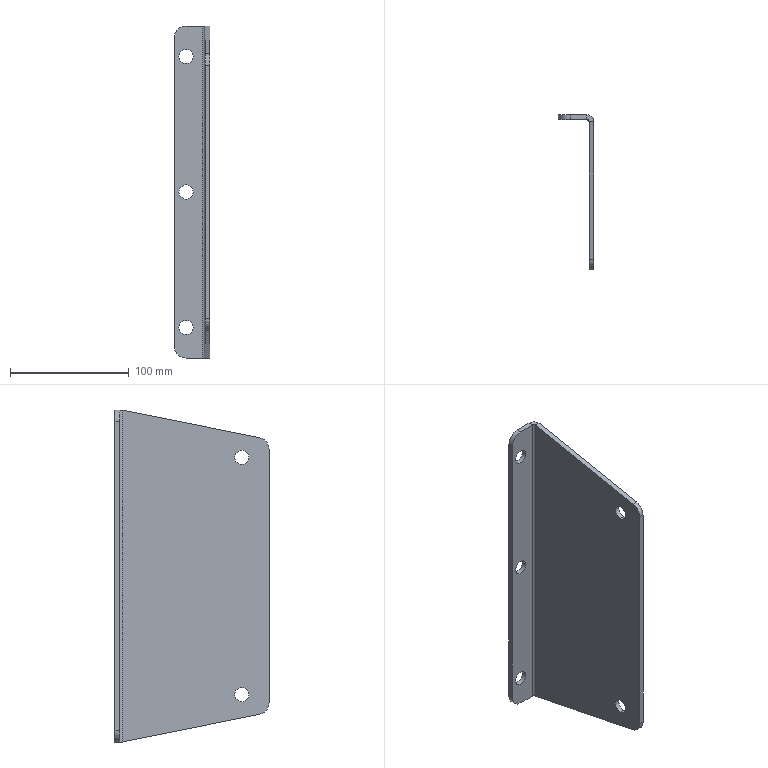Component | SolidWorks | JGS01-0004DriveFixingBracket-1 | 1 solid | 28 faces | box 30 x 130 x 280 mm | volume 157857 mm3 | cylinder 16 | plane 12 | commonest cylinder face diameters 12 x11 20 x4 4 x1 | material Plain Carbon Steel
STEP:
#1=COLOUR_RGB('',0.7922,0.8196,0.9333);
#2=FILL_AREA_STYLE_COLOUR('',#1);
#3=FILL_AREA_STYLE('',(#2));
#4=SURFACE_STYLE_FILL_AREA(#3);
#5=SURFACE_SIDE_STYLE('',(#4));
#6=SURFACE_STYLE_USAGE(.BOTH.,#5);
#7=PRESENTATION_STYLE_ASSIGNMENT((#6));
#8=CARTESIAN_POINT('',(-6.658,-2.86,5.951));
#9=VERTEX_POINT('',#8);
#10=CARTESIAN_POINT('',(-6.658,-2.86,6.423));
#11=VERTEX_POINT('',#10);
#12=CARTESIAN_POINT('',(-6.658,-2.86,6.187));
#13=DIRECTION('',(-1.,-0.,-0.));
#14=DIRECTION('',(0.,0.,1.));
#15=AXIS2_PLACEMENT_3D('',#12,#13,#14);
#16=CIRCLE('',#15,0.2362);
#17=EDGE_CURVE('',#9,#11,#16,.T.);
#18=ORIENTED_EDGE('',*,*,#17,.F.);
#19=CARTESIAN_POINT('',(-6.816,-2.86,5.951));
#20=VERTEX_POINT('',#19);
#21=CARTESIAN_POINT('',(-6.658,-2.86,5.951));
#22=DIRECTION('',(-1.,-0.,-0.));
#23=VECTOR('',#22,39.37);
#24=LINE('',#21,#23);
#25=EDGE_CURVE('',#9,#20,#24,.T.);
#26=ORIENTED_EDGE('',*,*,#25,.T.);
#27=CARTESIAN_POINT('',(-6.816,-2.86,6.423));
#28=VERTEX_POINT('',#27);
#29=CARTESIAN_POINT('',(-6.816,-2.86,6.187));
#30=DIRECTION('',(-1.,-0.,-0.));
#31=DIRECTION('',(0.,0.,1.));
#32=AXIS2_PLACEMENT_3D('',#29,#30,#31);
#33=CIRCLE('',#32,0.2362);
#34=EDGE_CURVE('',#20,#28,#33,.T.);
#35=ORIENTED_EDGE('',*,*,#34,.T.);
#36=CARTESIAN_POINT('',(-6.658,-2.86,6.423));
#37=DIRECTION('',(-1.,-0.,-0.));
#38=VECTOR('',#37,39.37);
#39=LINE('',#36,#38);
#40=EDGE_CURVE('',#11,#28,#39,.T.);
#41=ORIENTED_EDGE('',*,*,#40,.F.);
#42=EDGE_LOOP('',(#18,#26,#35,#41));
#43=FACE_OUTER_BOUND('',#42,.T.);
#44=CARTESIAN_POINT('',(-6.658,-2.86,6.187));
#45=DIRECTION('',(-1.,-0.,-0.));
#46=DIRECTION('',(0.,0.,1.));
#47=AXIS2_PLACEMENT_3D('',#44,#45,#46);
#48=CYLINDRICAL_SURFACE('',#47,0.2362);
#49=ADVANCED_FACE('',(#43),#48,.F.);
#50=CARTESIAN_POINT('',(-6.658,-2.86,-1.923));
#51=VERTEX_POINT('',#50);
#52=CARTESIAN_POINT('',(-6.658,-2.86,-1.451));
#53=VERTEX_POINT('',#52);
#54=CARTESIAN_POINT('',(-6.658,-2.86,-1.687));
#55=DIRECTION('',(-1.,-0.,-0.));
#56=DIRECTION('',(0.,0.,1.));
#57=AXIS2_PLACEMENT_3D('',#54,#55,#56);
#58=CIRCLE('',#57,0.2362);
#59=EDGE_CURVE('',#51,#53,#58,.T.);
#60=ORIENTED_EDGE('',*,*,#59,.F.);
#61=CARTESIAN_POINT('',(-6.816,-2.86,-1.923));
#62=VERTEX_POINT('',#61);
#63=CARTESIAN_POINT('',(-6.658,-2.86,-1.923));
#64=DIRECTION('',(-1.,-0.,-0.));
#65=VECTOR('',#64,39.37);
#66=LINE('',#63,#65);
#67=EDGE_CURVE('',#51,#62,#66,.T.);
#68=ORIENTED_EDGE('',*,*,#67,.T.);
#69=CARTESIAN_POINT('',(-6.816,-2.86,-1.451));
#70=VERTEX_POINT('',#69);
#71=CARTESIAN_POINT('',(-6.816,-2.86,-1.687));
#72=DIRECTION('',(-1.,-0.,-0.));
#73=DIRECTION('',(0.,0.,1.));
#74=AXIS2_PLACEMENT_3D('',#71,#72,#73);
#75=CIRCLE('',#74,0.2362);
#76=EDGE_CURVE('',#62,#70,#75,.T.);
#77=ORIENTED_EDGE('',*,*,#76,.T.);
#78=CARTESIAN_POINT('',(-6.658,-2.86,-1.451));
#79=DIRECTION('',(-1.,-0.,-0.));
#80=VECTOR('',#79,39.37);
#81=LINE('',#78,#80);
#82=EDGE_CURVE('',#53,#70,#81,.T.);
#83=ORIENTED_EDGE('',*,*,#82,.F.);
#84=EDGE_LOOP('',(#60,#68,#77,#83));
#85=FACE_OUTER_BOUND('',#84,.T.);
#86=CARTESIAN_POINT('',(-6.658,-2.86,-1.687));
#87=DIRECTION('',(-1.,-0.,-0.));
#88=DIRECTION('',(0.,0.,1.));
#89=AXIS2_PLACEMENT_3D('',#86,#87,#88);
#90=CYLINDRICAL_SURFACE('',#89,0.2362);
#91=ADVANCED_FACE('',(#85),#90,.F.);
#92=CARTESIAN_POINT('',(-7.682,1.196,2.25));
#93=VERTEX_POINT('',#92);
#94=CARTESIAN_POINT('',(-7.209,1.196,2.25));
#95=VERTEX_POINT('',#94);
#96=CARTESIAN_POINT('',(-7.446,1.196,2.25));
#97=DIRECTION('',(-0.,1.,-0.));
#98=DIRECTION('',(1.,0.,0.));
#99=AXIS2_PLACEMENT_3D('',#96,#97,#98);
#100=CIRCLE('',#99,0.2362);
#101=EDGE_CURVE('',#93,#95,#100,.T.);
#102=ORIENTED_EDGE('',*,*,#101,.F.);
#103=CARTESIAN_POINT('',(-7.682,1.353,2.25));
#104=VERTEX_POINT('',#103);
#105=CARTESIAN_POINT('',(-7.682,1.196,2.25));
#106=DIRECTION('',(-0.,1.,-0.));
#107=VECTOR('',#106,39.37);
#108=LINE('',#105,#107);
#109=EDGE_CURVE('',#93,#104,#108,.T.);
#110=ORIENTED_EDGE('',*,*,#109,.T.);
#111=CARTESIAN_POINT('',(-7.209,1.353,2.25));
#112=VERTEX_POINT('',#111);
#113=CARTESIAN_POINT('',(-7.446,1.353,2.25));
#114=DIRECTION('',(-0.,1.,-0.));
#115=DIRECTION('',(1.,0.,0.));
#116=AXIS2_PLACEMENT_3D('',#113,#114,#115);
#117=CIRCLE('',#116,0.2362);
#118=EDGE_CURVE('',#104,#112,#117,.T.);
#119=ORIENTED_EDGE('',*,*,#118,.T.);
#120=CARTESIAN_POINT('',(-7.209,1.196,2.25));
#121=DIRECTION('',(-0.,1.,-0.));
#122=VECTOR('',#121,39.37);
#123=LINE('',#120,#122);
#124=EDGE_CURVE('',#95,#112,#123,.T.);
#125=ORIENTED_EDGE('',*,*,#124,.F.);
#126=EDGE_LOOP('',(#102,#110,#119,#125));
#127=FACE_OUTER_BOUND('',#126,.T.);
#128=CARTESIAN_POINT('',(-7.446,1.196,2.25));
#129=DIRECTION('',(-0.,1.,-0.));
#130=DIRECTION('',(1.,0.,0.));
#131=AXIS2_PLACEMENT_3D('',#128,#129,#130);
#132=CYLINDRICAL_SURFACE('',#131,0.2362);
#133=ADVANCED_FACE('',(#127),#132,.F.);
#134=CARTESIAN_POINT('',(-7.682,1.196,-2.25));
#135=VERTEX_POINT('',#134);
#136=CARTESIAN_POINT('',(-7.209,1.196,-2.25));
#137=VERTEX_POINT('',#136);
#138=CARTESIAN_POINT('',(-7.446,1.196,-2.25));
#139=DIRECTION('',(-0.,1.,-0.));
#140=DIRECTION('',(1.,0.,0.));
#141=AXIS2_PLACEMENT_3D('',#138,#139,#140);
#142=CIRCLE('',#141,0.2362);
#143=EDGE_CURVE('',#135,#137,#142,.T.);
#144=ORIENTED_EDGE('',*,*,#143,.F.);
#145=CARTESIAN_POINT('',(-7.682,1.353,-2.25));
#146=VERTEX_POINT('',#145);
#147=CARTESIAN_POINT('',(-7.682,1.196,-2.25));
#148=DIRECTION('',(-0.,1.,-0.));
#149=VECTOR('',#148,39.37);
#150=LINE('',#147,#149);
#151=EDGE_CURVE('',#135,#146,#150,.T.);
#152=ORIENTED_EDGE('',*,*,#151,.T.);
#153=CARTESIAN_POINT('',(-7.209,1.353,-2.25));
#154=VERTEX_POINT('',#153);
#155=CARTESIAN_POINT('',(-7.446,1.353,-2.25));
#156=DIRECTION('',(-0.,1.,-0.));
#157=DIRECTION('',(1.,0.,0.));
#158=AXIS2_PLACEMENT_3D('',#155,#156,#157);
#159=CIRCLE('',#158,0.2362);
#160=EDGE_CURVE('',#146,#154,#159,.T.);
#161=ORIENTED_EDGE('',*,*,#160,.T.);
#162=CARTESIAN_POINT('',(-7.209,1.196,-2.25));
#163=DIRECTION('',(-0.,1.,-0.));
#164=VECTOR('',#163,39.37);
#165=LINE('',#162,#164);
#166=EDGE_CURVE('',#137,#154,#165,.T.);
#167=ORIENTED_EDGE('',*,*,#166,.F.);
#168=EDGE_LOOP('',(#144,#152,#161,#167));
#169=FACE_OUTER_BOUND('',#168,.T.);
#170=CARTESIAN_POINT('',(-7.446,1.196,-2.25));
#171=DIRECTION('',(-0.,1.,-0.));
#172=DIRECTION('',(1.,0.,0.));
#173=AXIS2_PLACEMENT_3D('',#170,#171,#172);
#174=CYLINDRICAL_SURFACE('',#173,0.2362);
#175=ADVANCED_FACE('',(#169),#174,.F.);
#176=CARTESIAN_POINT('',(-7.682,1.196,6.75));
#177=VERTEX_POINT('',#176);
#178=CARTESIAN_POINT('',(-7.209,1.196,6.75));
#179=VERTEX_POINT('',#178);
#180=CARTESIAN_POINT('',(-7.446,1.196,6.75));
#181=DIRECTION('',(-0.,1.,-0.));
#182=DIRECTION('',(1.,0.,0.));
#183=AXIS2_PLACEMENT_3D('',#180,#181,#182);
#184=CIRCLE('',#183,0.2362);
#185=EDGE_CURVE('',#177,#179,#184,.T.);
#186=ORIENTED_EDGE('',*,*,#185,.F.);
#187=CARTESIAN_POINT('',(-7.682,1.353,6.75));
#188=VERTEX_POINT('',#187);
#189=CARTESIAN_POINT('',(-7.682,1.196,6.75));
#190=DIRECTION('',(-0.,1.,-0.));
#191=VECTOR('',#190,39.37);
#192=LINE('',#189,#191);
#193=EDGE_CURVE('',#177,#188,#192,.T.);
#194=ORIENTED_EDGE('',*,*,#193,.T.);
#195=CARTESIAN_POINT('',(-7.209,1.353,6.75));
#196=VERTEX_POINT('',#195);
#197=CARTESIAN_POINT('',(-7.446,1.353,6.75));
#198=DIRECTION('',(-0.,1.,-0.));
#199=DIRECTION('',(1.,0.,0.));
#200=AXIS2_PLACEMENT_3D('',#197,#198,#199);
#201=CIRCLE('',#200,0.2362);
#202=EDGE_CURVE('',#188,#196,#201,.T.);
#203=ORIENTED_EDGE('',*,*,#202,.T.);
#204=CARTESIAN_POINT('',(-7.209,1.196,6.75));
#205=DIRECTION('',(-0.,1.,-0.));
#206=VECTOR('',#205,39.37);
#207=LINE('',#204,#206);
#208=EDGE_CURVE('',#179,#196,#207,.T.);
#209=ORIENTED_EDGE('',*,*,#208,.F.);
#210=EDGE_LOOP('',(#186,#194,#203,#209));
#211=FACE_OUTER_BOUND('',#210,.T.);
#212=CARTESIAN_POINT('',(-7.446,1.196,6.75));
#213=DIRECTION('',(-0.,1.,-0.));
#214=DIRECTION('',(1.,0.,0.));
#215=AXIS2_PLACEMENT_3D('',#212,#213,#214);
#216=CYLINDRICAL_SURFACE('',#215,0.2362);
#217=ADVANCED_FACE('',(#211),#216,.F.);
#218=CARTESIAN_POINT('',(-6.816,-2.86,6.187));
#219=DIRECTION('',(-1.,-0.,-0.));
#220=DIRECTION('',(0.,0.,1.));
#221=AXIS2_PLACEMENT_3D('',#218,#219,#220);
#222=CIRCLE('',#221,0.2362);
#223=EDGE_CURVE('',#28,#20,#222,.T.);
#224=ORIENTED_EDGE('',*,*,#223,.F.);
#225=ORIENTED_EDGE('',*,*,#34,.F.);
#226=EDGE_LOOP('',(#224,#225));
#227=FACE_BOUND('',#226,.T.);
#228=CARTESIAN_POINT('',(-6.816,-2.86,-1.687));
#229=DIRECTION('',(-1.,-0.,-0.));
#230=DIRECTION('',(0.,0.,1.));
#231=AXIS2_PLACEMENT_3D('',#228,#229,#230);
#232=CIRCLE('',#231,0.2362);
#233=EDGE_CURVE('',#70,#62,#232,.T.);
#234=ORIENTED_EDGE('',*,*,#233,.F.);
#235=ORIENTED_EDGE('',*,*,#76,.F.);
#236=EDGE_LOOP('',(#234,#235));
#237=FACE_BOUND('',#236,.T.);
#238=CARTESIAN_POINT('',(-6.816,1.117,-3.262));
#239=VERTEX_POINT('',#238);
#240=CARTESIAN_POINT('',(-6.816,-3.449,-2.341));
#241=VERTEX_POINT('',#240);
#242=CARTESIAN_POINT('',(-6.816,1.117,-3.262));
#243=DIRECTION('',(0.,-0.9803,0.1976));
#244=VECTOR('',#243,39.37);
#245=LINE('',#242,#244);
#246=EDGE_CURVE('',#239,#241,#245,.T.);
#247=ORIENTED_EDGE('',*,*,#246,.T.);
#248=CARTESIAN_POINT('',(-6.816,-3.765,-1.955));
#249=VERTEX_POINT('',#248);
#250=CARTESIAN_POINT('',(-6.816,-3.371,-1.955));
#251=DIRECTION('',(-1.,-0.,-0.));
#252=DIRECTION('',(0.,0.,1.));
#253=AXIS2_PLACEMENT_3D('',#250,#251,#252);
#254=CIRCLE('',#253,0.3937);
#255=EDGE_CURVE('',#241,#249,#254,.T.);
#256=ORIENTED_EDGE('',*,*,#255,.T.);
#257=CARTESIAN_POINT('',(-6.816,-3.765,6.455));
#258=VERTEX_POINT('',#257);
#259=CARTESIAN_POINT('',(-6.816,-3.765,7.762));
#260=DIRECTION('',(0.,0.,-1.));
#261=VECTOR('',#260,39.37);
#262=LINE('',#259,#261);
#263=EDGE_CURVE('',#258,#249,#262,.T.);
#264=ORIENTED_EDGE('',*,*,#263,.F.);
#265=CARTESIAN_POINT('',(-6.816,-3.449,6.841));
#266=VERTEX_POINT('',#265);
#267=CARTESIAN_POINT('',(-6.816,-3.371,6.455));
#268=DIRECTION('',(-1.,-0.,-0.));
#269=DIRECTION('',(0.,0.,1.));
#270=AXIS2_PLACEMENT_3D('',#267,#268,#269);
#271=CIRCLE('',#270,0.3937);
#272=EDGE_CURVE('',#258,#266,#271,.T.);
#273=ORIENTED_EDGE('',*,*,#272,.T.);
#274=CARTESIAN_POINT('',(-6.816,1.117,7.762));
#275=VERTEX_POINT('',#274);
#276=CARTESIAN_POINT('',(-6.816,-3.765,6.778));
#277=DIRECTION('',(-0.,0.9803,0.1976));
#278=VECTOR('',#277,39.37);
#279=LINE('',#276,#278);
#280=EDGE_CURVE('',#266,#275,#279,.T.);
#281=ORIENTED_EDGE('',*,*,#280,.T.);
#282=CARTESIAN_POINT('',(-6.816,1.117,-3.262));
#283=DIRECTION('',(-0.,-0.,1.));
#284=VECTOR('',#283,39.37);
#285=LINE('',#282,#284);
#286=EDGE_CURVE('',#239,#275,#285,.T.);
#287=ORIENTED_EDGE('',*,*,#286,.F.);
#288=EDGE_LOOP('',(#247,#256,#264,#273,#281,#287));
#289=FACE_OUTER_BOUND('',#288,.T.);
#290=CARTESIAN_POINT('',(-6.816,-1.206,2.25));
#291=DIRECTION('',(-1.,-0.,-0.));
#292=DIRECTION('',(-0.,-0.,1.));
#293=AXIS2_PLACEMENT_3D('',#290,#291,#292);
#294=PLANE('',#293);
#295=ADVANCED_FACE('',(#227,#237,#289),#294,.T.);
#296=CARTESIAN_POINT('',(-6.658,-2.86,6.187));
#297=DIRECTION('',(-1.,-0.,-0.));
#298=DIRECTION('',(0.,0.,1.));
#299=AXIS2_PLACEMENT_3D('',#296,#297,#298);
#300=CIRCLE('',#299,0.2362);
#301=EDGE_CURVE('',#11,#9,#300,.T.);
#302=ORIENTED_EDGE('',*,*,#301,.T.);
#303=ORIENTED_EDGE('',*,*,#17,.T.);
#304=EDGE_LOOP('',(#302,#303));
#305=FACE_BOUND('',#304,.T.);
#306=CARTESIAN_POINT('',(-6.658,-2.86,-1.687));
#307=DIRECTION('',(-1.,-0.,-0.));
#308=DIRECTION('',(0.,0.,1.));
#309=AXIS2_PLACEMENT_3D('',#306,#307,#308);
#310=CIRCLE('',#309,0.2362);
#311=EDGE_CURVE('',#53,#51,#310,.T.);
#312=ORIENTED_EDGE('',*,*,#311,.T.);
#313=ORIENTED_EDGE('',*,*,#59,.T.);
#314=EDGE_LOOP('',(#312,#313));
#315=FACE_BOUND('',#314,.T.);
#316=CARTESIAN_POINT('',(-6.658,-3.765,6.455));
#317=VERTEX_POINT('',#316);
#318=CARTESIAN_POINT('',(-6.658,-3.765,-1.955));
#319=VERTEX_POINT('',#318);
#320=CARTESIAN_POINT('',(-6.658,-3.765,7.762));
#321=DIRECTION('',(0.,0.,-1.));
#322=VECTOR('',#321,39.37);
#323=LINE('',#320,#322);
#324=EDGE_CURVE('',#317,#319,#323,.T.);
#325=ORIENTED_EDGE('',*,*,#324,.T.);
#326=CARTESIAN_POINT('',(-6.658,-3.449,-2.341));
#327=VERTEX_POINT('',#326);
#328=CARTESIAN_POINT('',(-6.658,-3.371,-1.955));
#329=DIRECTION('',(1.,0.,0.));
#330=DIRECTION('',(0.,0.,1.));
#331=AXIS2_PLACEMENT_3D('',#328,#329,#330);
#332=CIRCLE('',#331,0.3937);
#333=EDGE_CURVE('',#319,#327,#332,.T.);
#334=ORIENTED_EDGE('',*,*,#333,.T.);
#335=CARTESIAN_POINT('',(-6.658,1.117,-3.262));
#336=VERTEX_POINT('',#335);
#337=CARTESIAN_POINT('',(-6.658,1.117,-3.262));
#338=DIRECTION('',(0.,-0.9803,0.1976));
#339=VECTOR('',#338,39.37);
#340=LINE('',#337,#339);
#341=EDGE_CURVE('',#336,#327,#340,.T.);
#342=ORIENTED_EDGE('',*,*,#341,.F.);
#343=CARTESIAN_POINT('',(-6.658,1.117,7.762));
#344=VERTEX_POINT('',#343);
#345=CARTESIAN_POINT('',(-6.658,1.117,-3.262));
#346=DIRECTION('',(-0.,-0.,1.));
#347=VECTOR('',#346,39.37);
#348=LINE('',#345,#347);
#349=EDGE_CURVE('',#336,#344,#348,.T.);
#350=ORIENTED_EDGE('',*,*,#349,.T.);
#351=CARTESIAN_POINT('',(-6.658,-3.449,6.841));
#352=VERTEX_POINT('',#351);
#353=CARTESIAN_POINT('',(-6.658,-3.765,6.778));
#354=DIRECTION('',(-0.,0.9803,0.1976));
#355=VECTOR('',#354,39.37);
#356=LINE('',#353,#355);
#357=EDGE_CURVE('',#352,#344,#356,.T.);
#358=ORIENTED_EDGE('',*,*,#357,.F.);
#359=CARTESIAN_POINT('',(-6.658,-3.371,6.455));
#360=DIRECTION('',(1.,0.,0.));
#361=DIRECTION('',(0.,-0.,1.));
#362=AXIS2_PLACEMENT_3D('',#359,#360,#361);
#363=CIRCLE('',#362,0.3937);
#364=EDGE_CURVE('',#352,#317,#363,.T.);
#365=ORIENTED_EDGE('',*,*,#364,.T.);
#366=EDGE_LOOP('',(#325,#334,#342,#350,#358,#365));
#367=FACE_OUTER_BOUND('',#366,.T.);
#368=CARTESIAN_POINT('',(-6.658,-1.206,2.25));
#369=DIRECTION('',(-1.,-0.,-0.));
#370=DIRECTION('',(-0.,-0.,1.));
#371=AXIS2_PLACEMENT_3D('',#368,#369,#370);
#372=PLANE('',#371);
#373=ADVANCED_FACE('',(#305,#315,#367),#372,.F.);
#374=ORIENTED_EDGE('',*,*,#263,.T.);
#375=CARTESIAN_POINT('',(-6.816,-3.765,-1.955));
#376=DIRECTION('',(1.,0.,0.));
#377=VECTOR('',#376,39.37);
#378=LINE('',#375,#377);
#379=EDGE_CURVE('',#249,#319,#378,.T.);
#380=ORIENTED_EDGE('',*,*,#379,.T.);
#381=ORIENTED_EDGE('',*,*,#324,.F.);
#382=CARTESIAN_POINT('',(-6.816,-3.765,6.455));
#383=DIRECTION('',(-1.,-0.,-0.));
#384=VECTOR('',#383,39.37);
#385=LINE('',#382,#384);
#386=EDGE_CURVE('',#317,#258,#385,.T.);
#387=ORIENTED_EDGE('',*,*,#386,.T.);
#388=EDGE_LOOP('',(#374,#380,#381,#387));
#389=FACE_OUTER_BOUND('',#388,.T.);
#390=CARTESIAN_POINT('',(-6.816,-3.765,7.762));
#391=DIRECTION('',(0.,-1.,0.));
#392=DIRECTION('',(-1.,-0.,-0.));
#393=AXIS2_PLACEMENT_3D('',#390,#391,#392);
#394=PLANE('',#393);
#395=ADVANCED_FACE('',(#389),#394,.T.);
#396=CARTESIAN_POINT('',(-6.894,1.196,7.762));
#397=VERTEX_POINT('',#396);
#398=CARTESIAN_POINT('',(-6.894,1.353,7.762));
#399=VERTEX_POINT('',#398);
#400=CARTESIAN_POINT('',(-6.894,1.353,7.762));
#401=DIRECTION('',(-0.,1.,-0.));
#402=VECTOR('',#401,39.37);
#403=LINE('',#400,#402);
#404=EDGE_CURVE('',#397,#399,#403,.T.);
#405=ORIENTED_EDGE('',*,*,#404,.F.);
#406=CARTESIAN_POINT('',(-6.894,1.117,7.762));
#407=DIRECTION('',(-0.,-0.,1.));
#408=DIRECTION('',(-1.,-0.,0.));
#409=AXIS2_PLACEMENT_3D('',#406,#407,#408);
#410=CIRCLE('',#409,0.07874);
#411=EDGE_CURVE('',#275,#397,#410,.T.);
#412=ORIENTED_EDGE('',*,*,#411,.F.);
#413=CARTESIAN_POINT('',(-6.816,1.117,7.762));
#414=DIRECTION('',(1.,0.,0.));
#415=VECTOR('',#414,39.37);
#416=LINE('',#413,#415);
#417=EDGE_CURVE('',#275,#344,#416,.T.);
#418=ORIENTED_EDGE('',*,*,#417,.T.);
#419=CARTESIAN_POINT('',(-6.894,1.117,7.762));
#420=DIRECTION('',(-0.,-0.,1.));
#421=DIRECTION('',(-1.,-0.,0.));
#422=AXIS2_PLACEMENT_3D('',#419,#420,#421);
#423=CIRCLE('',#422,0.2362);
#424=EDGE_CURVE('',#344,#399,#423,.T.);
#425=ORIENTED_EDGE('',*,*,#424,.T.);
#426=EDGE_LOOP('',(#405,#412,#418,#425));
#427=FACE_OUTER_BOUND('',#426,.T.);
#428=CARTESIAN_POINT('',(-6.894,1.117,7.762));
#429=DIRECTION('',(-0.,-0.,1.));
#430=DIRECTION('',(1.,0.,0.));
#431=AXIS2_PLACEMENT_3D('',#428,#429,#430);
#432=PLANE('',#431);
#433=ADVANCED_FACE('',(#427),#432,.T.);
#434=CARTESIAN_POINT('',(-6.894,1.196,-3.262));
#435=VERTEX_POINT('',#434);
#436=CARTESIAN_POINT('',(-6.894,1.117,-3.262));
#437=DIRECTION('',(0.,0.,-1.));
#438=DIRECTION('',(-1.,-0.,0.));
#439=AXIS2_PLACEMENT_3D('',#436,#437,#438);
#440=CIRCLE('',#439,0.07874);
#441=EDGE_CURVE('',#435,#239,#440,.T.);
#442=ORIENTED_EDGE('',*,*,#441,.F.);
#443=CARTESIAN_POINT('',(-6.894,1.353,-3.262));
#444=VERTEX_POINT('',#443);
#445=CARTESIAN_POINT('',(-6.894,1.196,-3.262));
#446=DIRECTION('',(-0.,1.,-0.));
#447=VECTOR('',#446,39.37);
#448=LINE('',#445,#447);
#449=EDGE_CURVE('',#435,#444,#448,.T.);
#450=ORIENTED_EDGE('',*,*,#449,.T.);
#451=CARTESIAN_POINT('',(-6.894,1.117,-3.262));
#452=DIRECTION('',(0.,0.,-1.));
#453=DIRECTION('',(-1.,-0.,0.));
#454=AXIS2_PLACEMENT_3D('',#451,#452,#453);
#455=CIRCLE('',#454,0.2362);
#456=EDGE_CURVE('',#444,#336,#455,.T.);
#457=ORIENTED_EDGE('',*,*,#456,.T.);
#458=CARTESIAN_POINT('',(-6.816,1.117,-3.262));
#459=DIRECTION('',(1.,0.,0.));
#460=VECTOR('',#459,39.37);
#461=LINE('',#458,#460);
#462=EDGE_CURVE('',#239,#336,#461,.T.);
#463=ORIENTED_EDGE('',*,*,#462,.F.);
#464=EDGE_LOOP('',(#442,#450,#457,#463));
#465=FACE_OUTER_BOUND('',#464,.T.);
#466=CARTESIAN_POINT('',(-6.894,1.117,-3.262));
#467=DIRECTION('',(-0.,-0.,1.));
#468=DIRECTION('',(1.,0.,0.));
#469=AXIS2_PLACEMENT_3D('',#466,#467,#468);
#470=PLANE('',#469);
#471=ADVANCED_FACE('',(#465),#470,.F.);
#472=ORIENTED_EDGE('',*,*,#349,.F.);
#473=ORIENTED_EDGE('',*,*,#456,.F.);
#474=CARTESIAN_POINT('',(-6.894,1.353,7.762));
#475=DIRECTION('',(-0.,-0.,1.));
#476=VECTOR('',#475,39.37);
#477=LINE('',#474,#476);
#478=EDGE_CURVE('',#444,#399,#477,.T.);
#479=ORIENTED_EDGE('',*,*,#478,.T.);
#480=ORIENTED_EDGE('',*,*,#424,.F.);
#481=EDGE_LOOP('',(#472,#473,#479,#480));
#482=FACE_OUTER_BOUND('',#481,.T.);
#483=CARTESIAN_POINT('',(-6.894,1.117,-3.262));
#484=DIRECTION('',(0.,0.,-1.));
#485=DIRECTION('',(0.,1.,0.));
#486=AXIS2_PLACEMENT_3D('',#483,#484,#485);
#487=CYLINDRICAL_SURFACE('',#486,0.2362);
#488=ADVANCED_FACE('',(#482),#487,.T.);
#489=ORIENTED_EDGE('',*,*,#286,.T.);
#490=ORIENTED_EDGE('',*,*,#411,.T.);
#491=CARTESIAN_POINT('',(-6.894,1.196,7.762));
#492=DIRECTION('',(0.,0.,-1.));
#493=VECTOR('',#492,39.37);
#494=LINE('',#491,#493);
#495=EDGE_CURVE('',#397,#435,#494,.T.);
#496=ORIENTED_EDGE('',*,*,#495,.T.);
#497=ORIENTED_EDGE('',*,*,#441,.T.);
#498=EDGE_LOOP('',(#489,#490,#496,#497));
#499=FACE_OUTER_BOUND('',#498,.T.);
#500=CARTESIAN_POINT('',(-6.894,1.117,-3.262));
#501=DIRECTION('',(0.,0.,-1.));
#502=DIRECTION('',(0.,1.,0.));
#503=AXIS2_PLACEMENT_3D('',#500,#501,#502);
#504=CYLINDRICAL_SURFACE('',#503,0.07874);
#505=ADVANCED_FACE('',(#499),#504,.F.);
#506=CARTESIAN_POINT('',(-7.446,1.196,-3.262));
#507=VERTEX_POINT('',#506);
#508=CARTESIAN_POINT('',(-7.839,1.196,-3.262));
#509=DIRECTION('',(-1.,-0.,-0.));
#510=VECTOR('',#509,39.37);
#511=LINE('',#508,#510);
#512=EDGE_CURVE('',#435,#507,#511,.T.);
#513=ORIENTED_EDGE('',*,*,#512,.T.);
#514=CARTESIAN_POINT('',(-7.446,1.353,-3.262));
#515=VERTEX_POINT('',#514);
#516=CARTESIAN_POINT('',(-7.446,1.353,-3.262));
#517=DIRECTION('',(-0.,1.,-0.));
#518=VECTOR('',#517,39.37);
#519=LINE('',#516,#518);
#520=EDGE_CURVE('',#507,#515,#519,.T.);
#521=ORIENTED_EDGE('',*,*,#520,.T.);
#522=CARTESIAN_POINT('',(-6.658,1.353,-3.262));
#523=DIRECTION('',(-1.,-0.,-0.));
#524=VECTOR('',#523,39.37);
#525=LINE('',#522,#524);
#526=EDGE_CURVE('',#444,#515,#525,.T.);
#527=ORIENTED_EDGE('',*,*,#526,.F.);
#528=ORIENTED_EDGE('',*,*,#449,.F.);
#529=EDGE_LOOP('',(#513,#521,#527,#528));
#530=FACE_OUTER_BOUND('',#529,.T.);
#531=CARTESIAN_POINT('',(-7.839,1.353,-3.262));
#532=DIRECTION('',(-0.,-0.,1.));
#533=DIRECTION('',(1.,0.,0.));
#534=AXIS2_PLACEMENT_3D('',#531,#532,#533);
#535=PLANE('',#534);
#536=ADVANCED_FACE('',(#530),#535,.F.);
#537=CARTESIAN_POINT('',(-7.446,1.353,7.762));
#538=VERTEX_POINT('',#537);
#539=CARTESIAN_POINT('',(-6.658,1.353,7.762));
#540=DIRECTION('',(1.,0.,0.));
#541=VECTOR('',#540,39.37);
#542=LINE('',#539,#541);
#543=EDGE_CURVE('',#538,#399,#542,.T.);
#544=ORIENTED_EDGE('',*,*,#543,.F.);
#545=CARTESIAN_POINT('',(-7.446,1.196,7.762));
#546=VERTEX_POINT('',#545);
#547=CARTESIAN_POINT('',(-7.446,1.353,7.762));
#548=DIRECTION('',(0.,-1.,0.));
#549=VECTOR('',#548,39.37);
#550=LINE('',#547,#549);
#551=EDGE_CURVE('',#538,#546,#550,.T.);
#552=ORIENTED_EDGE('',*,*,#551,.T.);
#553=CARTESIAN_POINT('',(-6.816,1.196,7.762));
#554=DIRECTION('',(1.,0.,0.));
#555=VECTOR('',#554,39.37);
#556=LINE('',#553,#555);
#557=EDGE_CURVE('',#546,#397,#556,.T.);
#558=ORIENTED_EDGE('',*,*,#557,.T.);
#559=ORIENTED_EDGE('',*,*,#404,.T.);
#560=EDGE_LOOP('',(#544,#552,#558,#559));
#561=FACE_OUTER_BOUND('',#560,.T.);
#562=CARTESIAN_POINT('',(-6.816,1.353,7.762));
#563=DIRECTION('',(0.,0.,-1.));
#564=DIRECTION('',(-1.,-0.,-0.));
#565=AXIS2_PLACEMENT_3D('',#562,#563,#564);
#566=PLANE('',#565);
#567=ADVANCED_FACE('',(#561),#566,.F.);
#568=CARTESIAN_POINT('',(-7.446,1.353,2.25));
#569=DIRECTION('',(-0.,1.,-0.));
#570=DIRECTION('',(1.,0.,0.));
#571=AXIS2_PLACEMENT_3D('',#568,#569,#570);
#572=CIRCLE('',#571,0.2362);
#573=EDGE_CURVE('',#112,#104,#572,.T.);
#574=ORIENTED_EDGE('',*,*,#573,.F.);
#575=ORIENTED_EDGE('',*,*,#118,.F.);
#576=EDGE_LOOP('',(#574,#575));
#577=FACE_BOUND('',#576,.T.);
#578=CARTESIAN_POINT('',(-7.446,1.353,-2.25));
#579=DIRECTION('',(-0.,1.,-0.));
#580=DIRECTION('',(1.,0.,0.));
#581=AXIS2_PLACEMENT_3D('',#578,#579,#580);
#582=CIRCLE('',#581,0.2362);
#583=EDGE_CURVE('',#154,#146,#582,.T.);
#584=ORIENTED_EDGE('',*,*,#583,.F.);
#585=ORIENTED_EDGE('',*,*,#160,.F.);
#586=EDGE_LOOP('',(#584,#585));
#587=FACE_BOUND('',#586,.T.);
#588=CARTESIAN_POINT('',(-7.446,1.353,6.75));
#589=DIRECTION('',(-0.,1.,-0.));
#590=DIRECTION('',(1.,0.,0.));
#591=AXIS2_PLACEMENT_3D('',#588,#589,#590);
#592=CIRCLE('',#591,0.2362);
#593=EDGE_CURVE('',#196,#188,#592,.T.);
#594=ORIENTED_EDGE('',*,*,#593,.F.);
#595=ORIENTED_EDGE('',*,*,#202,.F.);
#596=EDGE_LOOP('',(#594,#595));
#597=FACE_BOUND('',#596,.T.);
#598=CARTESIAN_POINT('',(-7.839,1.353,-2.868));
#599=VERTEX_POINT('',#598);
#600=CARTESIAN_POINT('',(-7.839,1.353,7.368));
#601=VERTEX_POINT('',#600);
#602=CARTESIAN_POINT('',(-7.839,1.353,2.25));
#603=DIRECTION('',(-0.,-0.,1.));
#604=VECTOR('',#603,39.37);
#605=LINE('',#602,#604);
#606=EDGE_CURVE('',#599,#601,#605,.T.);
#607=ORIENTED_EDGE('',*,*,#606,.T.);
#608=CARTESIAN_POINT('',(-7.446,1.353,7.368));
#609=DIRECTION('',(-0.,1.,-0.));
#610=DIRECTION('',(-1.,-0.,0.));
#611=AXIS2_PLACEMENT_3D('',#608,#609,#610);
#612=CIRCLE('',#611,0.3937);
#613=EDGE_CURVE('',#601,#538,#612,.T.);
#614=ORIENTED_EDGE('',*,*,#613,.T.);
#615=ORIENTED_EDGE('',*,*,#543,.T.);
#616=ORIENTED_EDGE('',*,*,#478,.F.);
#617=ORIENTED_EDGE('',*,*,#526,.T.);
#618=CARTESIAN_POINT('',(-7.446,1.353,-2.868));
#619=DIRECTION('',(-0.,1.,-0.));
#620=DIRECTION('',(-1.,-0.,0.));
#621=AXIS2_PLACEMENT_3D('',#618,#619,#620);
#622=CIRCLE('',#621,0.3937);
#623=EDGE_CURVE('',#515,#599,#622,.T.);
#624=ORIENTED_EDGE('',*,*,#623,.T.);
#625=EDGE_LOOP('',(#607,#614,#615,#616,#617,#624));
#626=FACE_OUTER_BOUND('',#625,.T.);
#627=CARTESIAN_POINT('',(-6.658,1.353,2.25));
#628=DIRECTION('',(0.,-1.,0.));
#629=DIRECTION('',(-1.,-0.,-0.));
#630=AXIS2_PLACEMENT_3D('',#627,#628,#629);
#631=PLANE('',#630);
#632=ADVANCED_FACE('',(#577,#587,#597,#626),#631,.F.);
#633=CARTESIAN_POINT('',(-7.446,1.196,2.25));
#634=DIRECTION('',(-0.,1.,-0.));
#635=DIRECTION('',(1.,0.,0.));
#636=AXIS2_PLACEMENT_3D('',#633,#634,#635);
#637=CIRCLE('',#636,0.2362);
#638=EDGE_CURVE('',#95,#93,#637,.T.);
#639=ORIENTED_EDGE('',*,*,#638,.T.);
#640=ORIENTED_EDGE('',*,*,#101,.T.);
#641=EDGE_LOOP('',(#639,#640));
#642=FACE_BOUND('',#641,.T.);
#643=CARTESIAN_POINT('',(-7.446,1.196,-2.25));
#644=DIRECTION('',(-0.,1.,-0.));
#645=DIRECTION('',(1.,0.,0.));
#646=AXIS2_PLACEMENT_3D('',#643,#644,#645);
#647=CIRCLE('',#646,0.2362);
#648=EDGE_CURVE('',#137,#135,#647,.T.);
#649=ORIENTED_EDGE('',*,*,#648,.T.);
#650=ORIENTED_EDGE('',*,*,#143,.T.);
#651=EDGE_LOOP('',(#649,#650));
#652=FACE_BOUND('',#651,.T.);
#653=CARTESIAN_POINT('',(-7.446,1.196,6.75));
#654=DIRECTION('',(-0.,1.,-0.));
#655=DIRECTION('',(1.,0.,0.));
#656=AXIS2_PLACEMENT_3D('',#653,#654,#655);
#657=CIRCLE('',#656,0.2362);
#658=EDGE_CURVE('',#179,#177,#657,.T.);
#659=ORIENTED_EDGE('',*,*,#658,.T.);
#660=ORIENTED_EDGE('',*,*,#185,.T.);
#661=EDGE_LOOP('',(#659,#660));
#662=FACE_BOUND('',#661,.T.);
#663=ORIENTED_EDGE('',*,*,#557,.F.);
#664=CARTESIAN_POINT('',(-7.839,1.196,7.368));
#665=VERTEX_POINT('',#664);
#666=CARTESIAN_POINT('',(-7.446,1.196,7.368));
#667=DIRECTION('',(0.,-1.,0.));
#668=DIRECTION('',(-1.,-0.,0.));
#669=AXIS2_PLACEMENT_3D('',#666,#667,#668);
#670=CIRCLE('',#669,0.3937);
#671=EDGE_CURVE('',#546,#665,#670,.T.);
#672=ORIENTED_EDGE('',*,*,#671,.T.);
#673=CARTESIAN_POINT('',(-7.839,1.196,-2.868));
#674=VERTEX_POINT('',#673);
#675=CARTESIAN_POINT('',(-7.839,1.196,7.762));
#676=DIRECTION('',(-0.,-0.,1.));
#677=VECTOR('',#676,39.37);
#678=LINE('',#675,#677);
#679=EDGE_CURVE('',#674,#665,#678,.T.);
#680=ORIENTED_EDGE('',*,*,#679,.F.);
#681=CARTESIAN_POINT('',(-7.446,1.196,-2.868));
#682=DIRECTION('',(0.,-1.,0.));
#683=DIRECTION('',(-1.,-0.,0.));
#684=AXIS2_PLACEMENT_3D('',#681,#682,#683);
#685=CIRCLE('',#684,0.3937);
#686=EDGE_CURVE('',#674,#507,#685,.T.);
#687=ORIENTED_EDGE('',*,*,#686,.T.);
#688=ORIENTED_EDGE('',*,*,#512,.F.);
#689=ORIENTED_EDGE('',*,*,#495,.F.);
#690=EDGE_LOOP('',(#663,#672,#680,#687,#688,#689));
#691=FACE_OUTER_BOUND('',#690,.T.);
#692=CARTESIAN_POINT('',(-6.658,1.196,2.25));
#693=DIRECTION('',(0.,-1.,0.));
#694=DIRECTION('',(-1.,-0.,-0.));
#695=AXIS2_PLACEMENT_3D('',#692,#693,#694);
#696=PLANE('',#695);
#697=ADVANCED_FACE('',(#642,#652,#662,#691),#696,.T.);
#698=ORIENTED_EDGE('',*,*,#679,.T.);
#699=CARTESIAN_POINT('',(-7.839,1.353,7.368));
#700=DIRECTION('',(-0.,1.,-0.));
#701=VECTOR('',#700,39.37);
#702=LINE('',#699,#701);
#703=EDGE_CURVE('',#665,#601,#702,.T.);
#704=ORIENTED_EDGE('',*,*,#703,.T.);
#705=ORIENTED_EDGE('',*,*,#606,.F.);
#706=CARTESIAN_POINT('',(-7.839,1.353,-2.868));
#707=DIRECTION('',(0.,-1.,0.));
#708=VECTOR('',#707,39.37);
#709=LINE('',#706,#708);
#710=EDGE_CURVE('',#599,#674,#709,.T.);
#711=ORIENTED_EDGE('',*,*,#710,.T.);
#712=EDGE_LOOP('',(#698,#704,#705,#711));
#713=FACE_OUTER_BOUND('',#712,.T.);
#714=CARTESIAN_POINT('',(-7.839,1.353,7.762));
#715=DIRECTION('',(1.,0.,0.));
#716=DIRECTION('',(0.,-1.,0.));
#717=AXIS2_PLACEMENT_3D('',#714,#715,#716);
#718=PLANE('',#717);
#719=ADVANCED_FACE('',(#713),#718,.F.);
#720=ORIENTED_EDGE('',*,*,#193,.F.);
#721=ORIENTED_EDGE('',*,*,#658,.F.);
#722=ORIENTED_EDGE('',*,*,#208,.T.);
#723=ORIENTED_EDGE('',*,*,#593,.T.);
#724=EDGE_LOOP('',(#720,#721,#722,#723));
#725=FACE_OUTER_BOUND('',#724,.T.);
#726=CARTESIAN_POINT('',(-7.446,1.196,6.75));
#727=DIRECTION('',(-0.,1.,-0.));
#728=DIRECTION('',(1.,0.,0.));
#729=AXIS2_PLACEMENT_3D('',#726,#727,#728);
#730=CYLINDRICAL_SURFACE('',#729,0.2362);
#731=ADVANCED_FACE('',(#725),#730,.F.);
#732=ORIENTED_EDGE('',*,*,#151,.F.);
#733=ORIENTED_EDGE('',*,*,#648,.F.);
#734=ORIENTED_EDGE('',*,*,#166,.T.);
#735=ORIENTED_EDGE('',*,*,#583,.T.);
#736=EDGE_LOOP('',(#732,#733,#734,#735));
#737=FACE_OUTER_BOUND('',#736,.T.);
#738=CARTESIAN_POINT('',(-7.446,1.196,-2.25));
#739=DIRECTION('',(-0.,1.,-0.));
#740=DIRECTION('',(1.,0.,0.));
#741=AXIS2_PLACEMENT_3D('',#738,#739,#740);
#742=CYLINDRICAL_SURFACE('',#741,0.2362);
#743=ADVANCED_FACE('',(#737),#742,.F.);
#744=ORIENTED_EDGE('',*,*,#109,.F.);
#745=ORIENTED_EDGE('',*,*,#638,.F.);
#746=ORIENTED_EDGE('',*,*,#124,.T.);
#747=ORIENTED_EDGE('',*,*,#573,.T.);
#748=EDGE_LOOP('',(#744,#745,#746,#747));
#749=FACE_OUTER_BOUND('',#748,.T.);
#750=CARTESIAN_POINT('',(-7.446,1.196,2.25));
#751=DIRECTION('',(-0.,1.,-0.));
#752=DIRECTION('',(1.,0.,0.));
#753=AXIS2_PLACEMENT_3D('',#750,#751,#752);
#754=CYLINDRICAL_SURFACE('',#753,0.2362);
#755=ADVANCED_FACE('',(#749),#754,.F.);
#756=ORIENTED_EDGE('',*,*,#67,.F.);
#757=ORIENTED_EDGE('',*,*,#311,.F.);
#758=ORIENTED_EDGE('',*,*,#82,.T.);
#759=ORIENTED_EDGE('',*,*,#233,.T.);
#760=EDGE_LOOP('',(#756,#757,#758,#759));
#761=FACE_OUTER_BOUND('',#760,.T.);
#762=CARTESIAN_POINT('',(-6.658,-2.86,-1.687));
#763=DIRECTION('',(-1.,-0.,-0.));
#764=DIRECTION('',(0.,0.,1.));
#765=AXIS2_PLACEMENT_3D('',#762,#763,#764);
#766=CYLINDRICAL_SURFACE('',#765,0.2362);
#767=ADVANCED_FACE('',(#761),#766,.F.);
#768=ORIENTED_EDGE('',*,*,#25,.F.);
#769=ORIENTED_EDGE('',*,*,#301,.F.);
#770=ORIENTED_EDGE('',*,*,#40,.T.);
#771=ORIENTED_EDGE('',*,*,#223,.T.);
#772=EDGE_LOOP('',(#768,#769,#770,#771));
#773=FACE_OUTER_BOUND('',#772,.T.);
#774=CARTESIAN_POINT('',(-6.658,-2.86,6.187));
#775=DIRECTION('',(-1.,-0.,-0.));
#776=DIRECTION('',(0.,0.,1.));
#777=AXIS2_PLACEMENT_3D('',#774,#775,#776);
#778=CYLINDRICAL_SURFACE('',#777,0.2362);
#779=ADVANCED_FACE('',(#773),#778,.F.);
#780=ORIENTED_EDGE('',*,*,#341,.T.);
#781=CARTESIAN_POINT('',(-6.658,-3.449,-2.341));
#782=DIRECTION('',(-1.,-0.,-0.));
#783=VECTOR('',#782,39.37);
#784=LINE('',#781,#783);
#785=EDGE_CURVE('',#327,#241,#784,.T.);
#786=ORIENTED_EDGE('',*,*,#785,.T.);
#787=ORIENTED_EDGE('',*,*,#246,.F.);
#788=ORIENTED_EDGE('',*,*,#462,.T.);
#789=EDGE_LOOP('',(#780,#786,#787,#788));
#790=FACE_OUTER_BOUND('',#789,.T.);
#791=CARTESIAN_POINT('',(-6.658,1.117,-3.262));
#792=DIRECTION('',(0.,-0.1976,-0.9803));
#793=DIRECTION('',(0.,-0.9803,0.1976));
#794=AXIS2_PLACEMENT_3D('',#791,#792,#793);
#795=PLANE('',#794);
#796=ADVANCED_FACE('',(#790),#795,.T.);
#797=ORIENTED_EDGE('',*,*,#280,.F.);
#798=CARTESIAN_POINT('',(-6.658,-3.449,6.841));
#799=DIRECTION('',(1.,0.,0.));
#800=VECTOR('',#799,39.37);
#801=LINE('',#798,#800);
#802=EDGE_CURVE('',#266,#352,#801,.T.);
#803=ORIENTED_EDGE('',*,*,#802,.T.);
#804=ORIENTED_EDGE('',*,*,#357,.T.);
#805=ORIENTED_EDGE('',*,*,#417,.F.);
#806=EDGE_LOOP('',(#797,#803,#804,#805));
#807=FACE_OUTER_BOUND('',#806,.T.);
#808=CARTESIAN_POINT('',(-6.658,-3.765,6.778));
#809=DIRECTION('',(0.,-0.1976,0.9803));
#810=DIRECTION('',(-0.,0.9803,0.1976));
#811=AXIS2_PLACEMENT_3D('',#808,#809,#810);
#812=PLANE('',#811);
#813=ADVANCED_FACE('',(#807),#812,.T.);
#814=ORIENTED_EDGE('',*,*,#333,.F.);
#815=ORIENTED_EDGE('',*,*,#379,.F.);
#816=ORIENTED_EDGE('',*,*,#255,.F.);
#817=ORIENTED_EDGE('',*,*,#785,.F.);
#818=EDGE_LOOP('',(#814,#815,#816,#817));
#819=FACE_OUTER_BOUND('',#818,.T.);
#820=CARTESIAN_POINT('',(-6.658,-3.371,-1.955));
#821=DIRECTION('',(-1.,-0.,-0.));
#822=DIRECTION('',(0.,0.,1.));
#823=AXIS2_PLACEMENT_3D('',#820,#821,#822);
#824=CYLINDRICAL_SURFACE('',#823,0.3937);
#825=ADVANCED_FACE('',(#819),#824,.T.);
#826=ORIENTED_EDGE('',*,*,#364,.F.);
#827=ORIENTED_EDGE('',*,*,#802,.F.);
#828=ORIENTED_EDGE('',*,*,#272,.F.);
#829=ORIENTED_EDGE('',*,*,#386,.F.);
#830=EDGE_LOOP('',(#826,#827,#828,#829));
#831=FACE_OUTER_BOUND('',#830,.T.);
#832=CARTESIAN_POINT('',(-6.816,-3.371,6.455));
#833=DIRECTION('',(-1.,-0.,-0.));
#834=DIRECTION('',(0.,0.,1.));
#835=AXIS2_PLACEMENT_3D('',#832,#833,#834);
#836=CYLINDRICAL_SURFACE('',#835,0.3937);
#837=ADVANCED_FACE('',(#831),#836,.T.);
#838=ORIENTED_EDGE('',*,*,#613,.F.);
#839=ORIENTED_EDGE('',*,*,#703,.F.);
#840=ORIENTED_EDGE('',*,*,#671,.F.);
#841=ORIENTED_EDGE('',*,*,#551,.F.);
#842=EDGE_LOOP('',(#838,#839,#840,#841));
#843=FACE_OUTER_BOUND('',#842,.T.);
#844=CARTESIAN_POINT('',(-7.446,1.353,7.368));
#845=DIRECTION('',(0.,-1.,0.));
#846=DIRECTION('',(-1.,-0.,0.));
#847=AXIS2_PLACEMENT_3D('',#844,#845,#846);
#848=CYLINDRICAL_SURFACE('',#847,0.3937);
#849=ADVANCED_FACE('',(#843),#848,.T.);
#850=ORIENTED_EDGE('',*,*,#623,.F.);
#851=ORIENTED_EDGE('',*,*,#520,.F.);
#852=ORIENTED_EDGE('',*,*,#686,.F.);
#853=ORIENTED_EDGE('',*,*,#710,.F.);
#854=EDGE_LOOP('',(#850,#851,#852,#853));
#855=FACE_OUTER_BOUND('',#854,.T.);
#856=CARTESIAN_POINT('',(-7.446,1.353,-2.868));
#857=DIRECTION('',(0.,-1.,0.));
#858=DIRECTION('',(-1.,-0.,0.));
#859=AXIS2_PLACEMENT_3D('',#856,#857,#858);
#860=CYLINDRICAL_SURFACE('',#859,0.3937);
#861=ADVANCED_FACE('',(#855),#860,.T.);
#862=CLOSED_SHELL('',(#49,#91,#133,#175,#217,#295,#373,#395,#433,#471,#488,#505,#536,#567,#632,#697,#719,#731,#743,#755,#767,#779,#796,#813,#825,#837,#849,#861));
#863=MANIFOLD_SOLID_BREP('',#862);
#864=STYLED_ITEM('',(#7),#863);
#865=PRESENTATION_LAYER_ASSIGNMENT('','',(#864));
#866=CARTESIAN_POINT('',(0.,0.,0.));
#867=DIRECTION('',(0.,0.,1.));
#868=DIRECTION('',(1.,0.,0.));
#869=AXIS2_PLACEMENT_3D('',#866,#867,#868);
#870=(LENGTH_UNIT()NAMED_UNIT(*)SI_UNIT($,.METRE.));
#871=LENGTH_MEASURE_WITH_UNIT(LENGTH_MEASURE(0.0254),#870);
#872=DIMENSIONAL_EXPONENTS(1.,0.,0.,0.,0.,0.,0.);
#873=(CONVERSION_BASED_UNIT('',#871)LENGTH_UNIT()NAMED_UNIT(#872));
#874=UNCERTAINTY_MEASURE_WITH_UNIT(LENGTH_MEASURE(0.00001),#873,'','');
#875=(NAMED_UNIT(*)PLANE_ANGLE_UNIT()SI_UNIT($,.RADIAN.));
#876=(NAMED_UNIT(*)SI_UNIT($,.STERADIAN.)SOLID_ANGLE_UNIT());
#877=(GEOMETRIC_REPRESENTATION_CONTEXT(3)GLOBAL_UNCERTAINTY_ASSIGNED_CONTEXT((#874))GLOBAL_UNIT_ASSIGNED_CONTEXT((#873,#875,#876))REPRESENTATION_CONTEXT('',''));
#878=ADVANCED_BREP_SHAPE_REPRESENTATION('',(#863,#869),#877);
#879=(LENGTH_UNIT()NAMED_UNIT(*)SI_UNIT($,.METRE.));
#880=LENGTH_MEASURE_WITH_UNIT(LENGTH_MEASURE(0.0254),#879);
#881=DIMENSIONAL_EXPONENTS(1.,0.,0.,0.,0.,0.,0.);
#882=(CONVERSION_BASED_UNIT('',#880)LENGTH_UNIT()NAMED_UNIT(#881));
#883=UNCERTAINTY_MEASURE_WITH_UNIT(LENGTH_MEASURE(0.00001),#882,'','');
#884=(NAMED_UNIT(*)PLANE_ANGLE_UNIT()SI_UNIT($,.RADIAN.));
#885=(NAMED_UNIT(*)SI_UNIT($,.STERADIAN.)SOLID_ANGLE_UNIT());
#886=(GEOMETRIC_REPRESENTATION_CONTEXT(3)GLOBAL_UNCERTAINTY_ASSIGNED_CONTEXT((#883))GLOBAL_UNIT_ASSIGNED_CONTEXT((#882,#884,#885))REPRESENTATION_CONTEXT('',''));
#887=MECHANICAL_DESIGN_GEOMETRIC_PRESENTATION_REPRESENTATION('',(#864),#886);